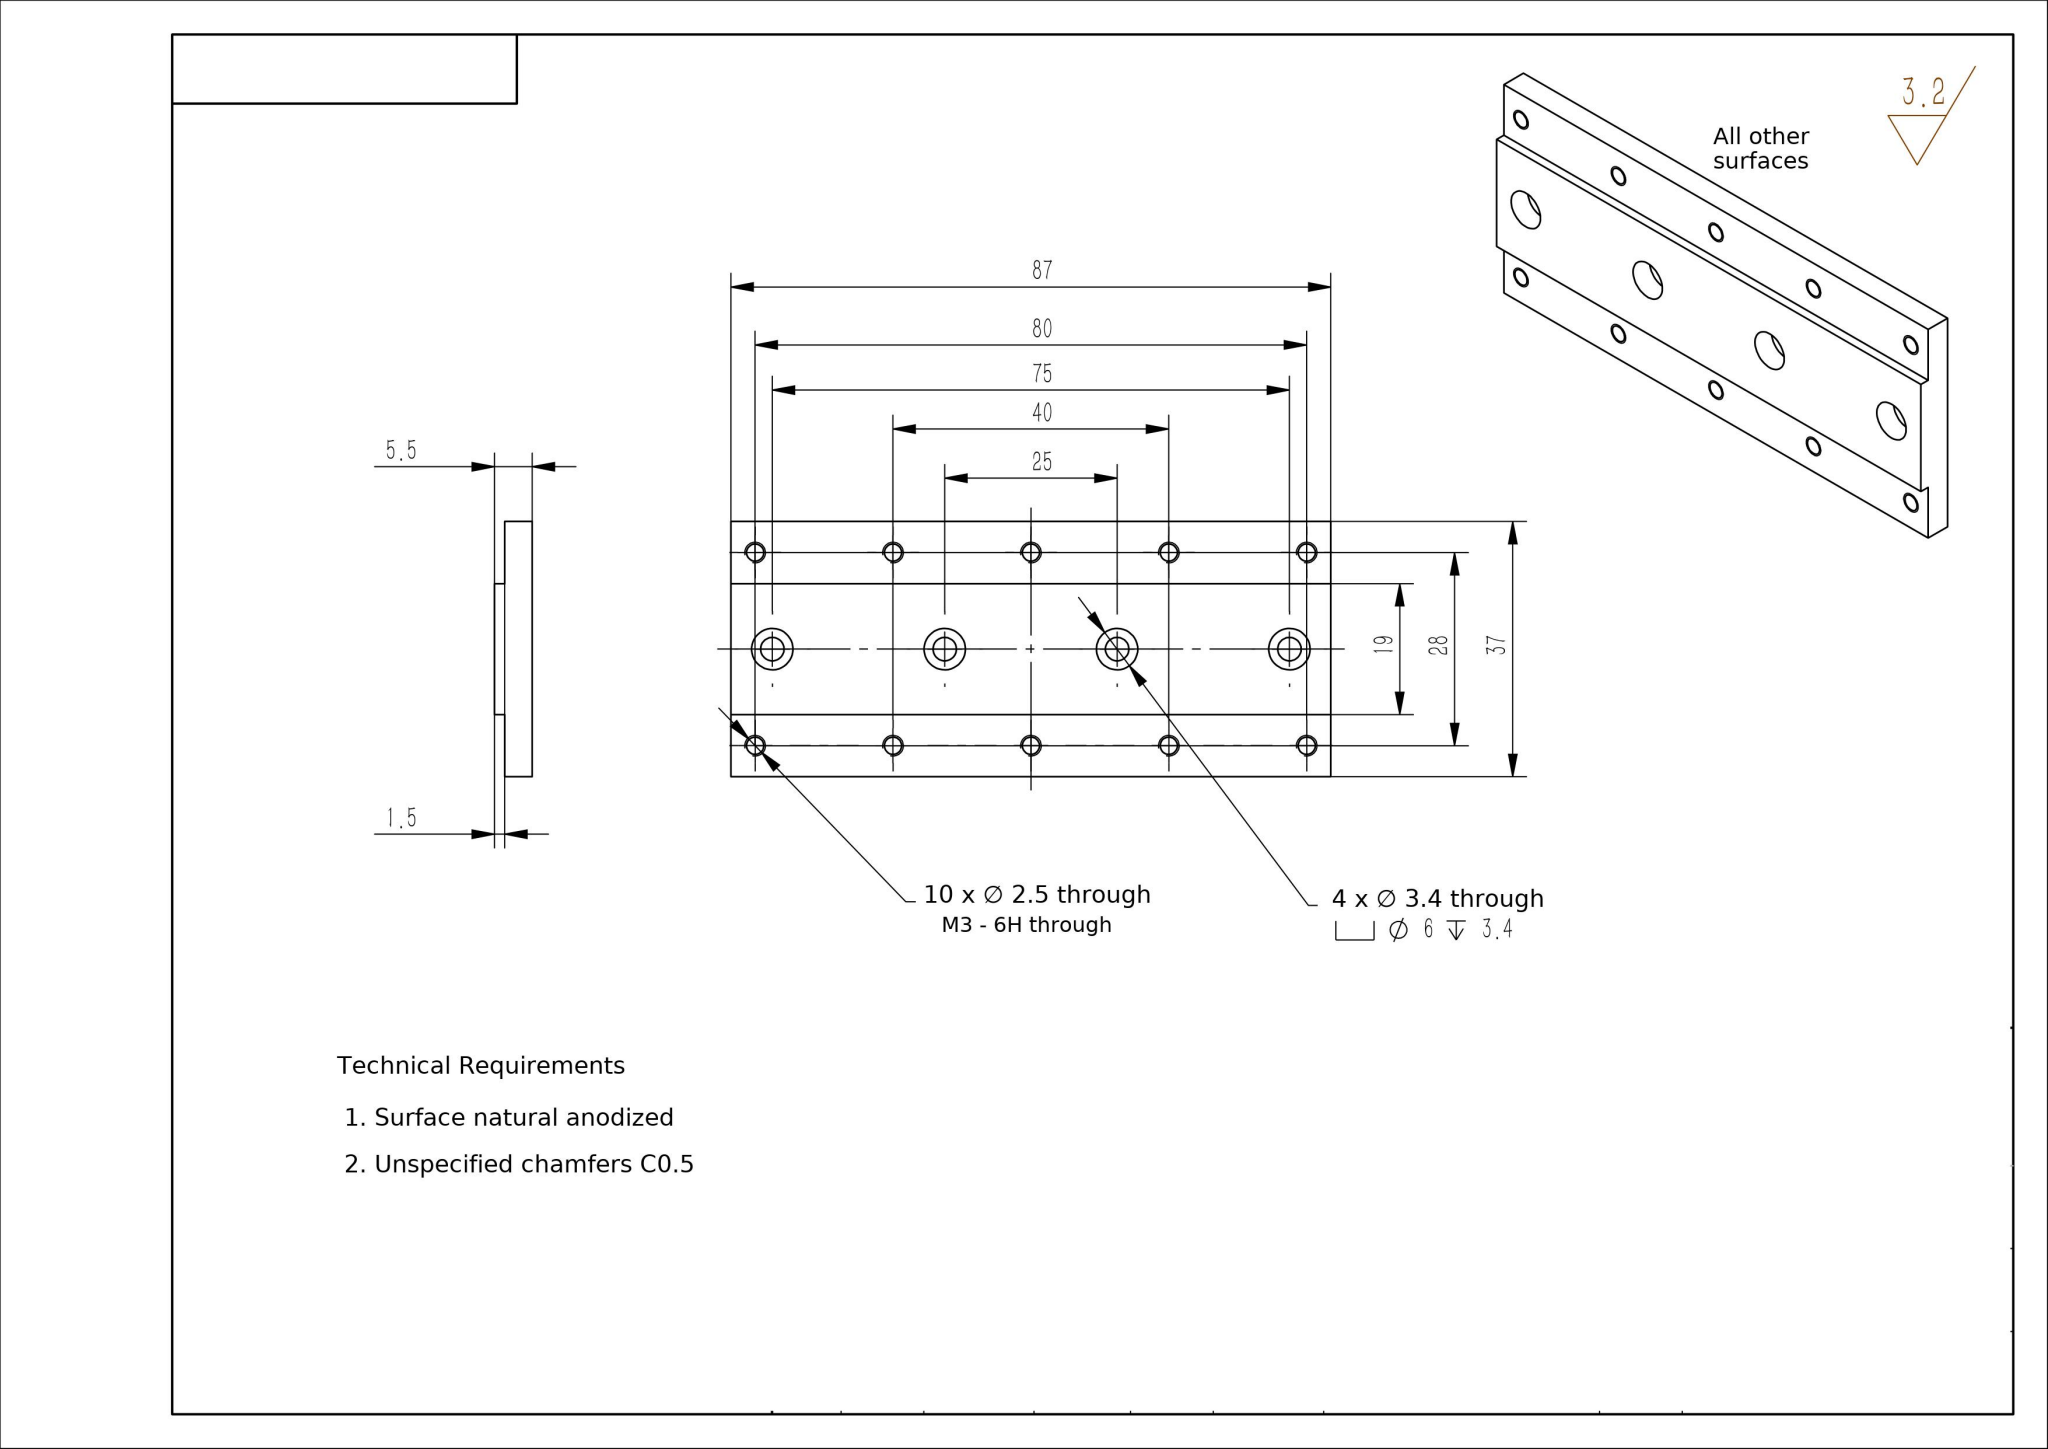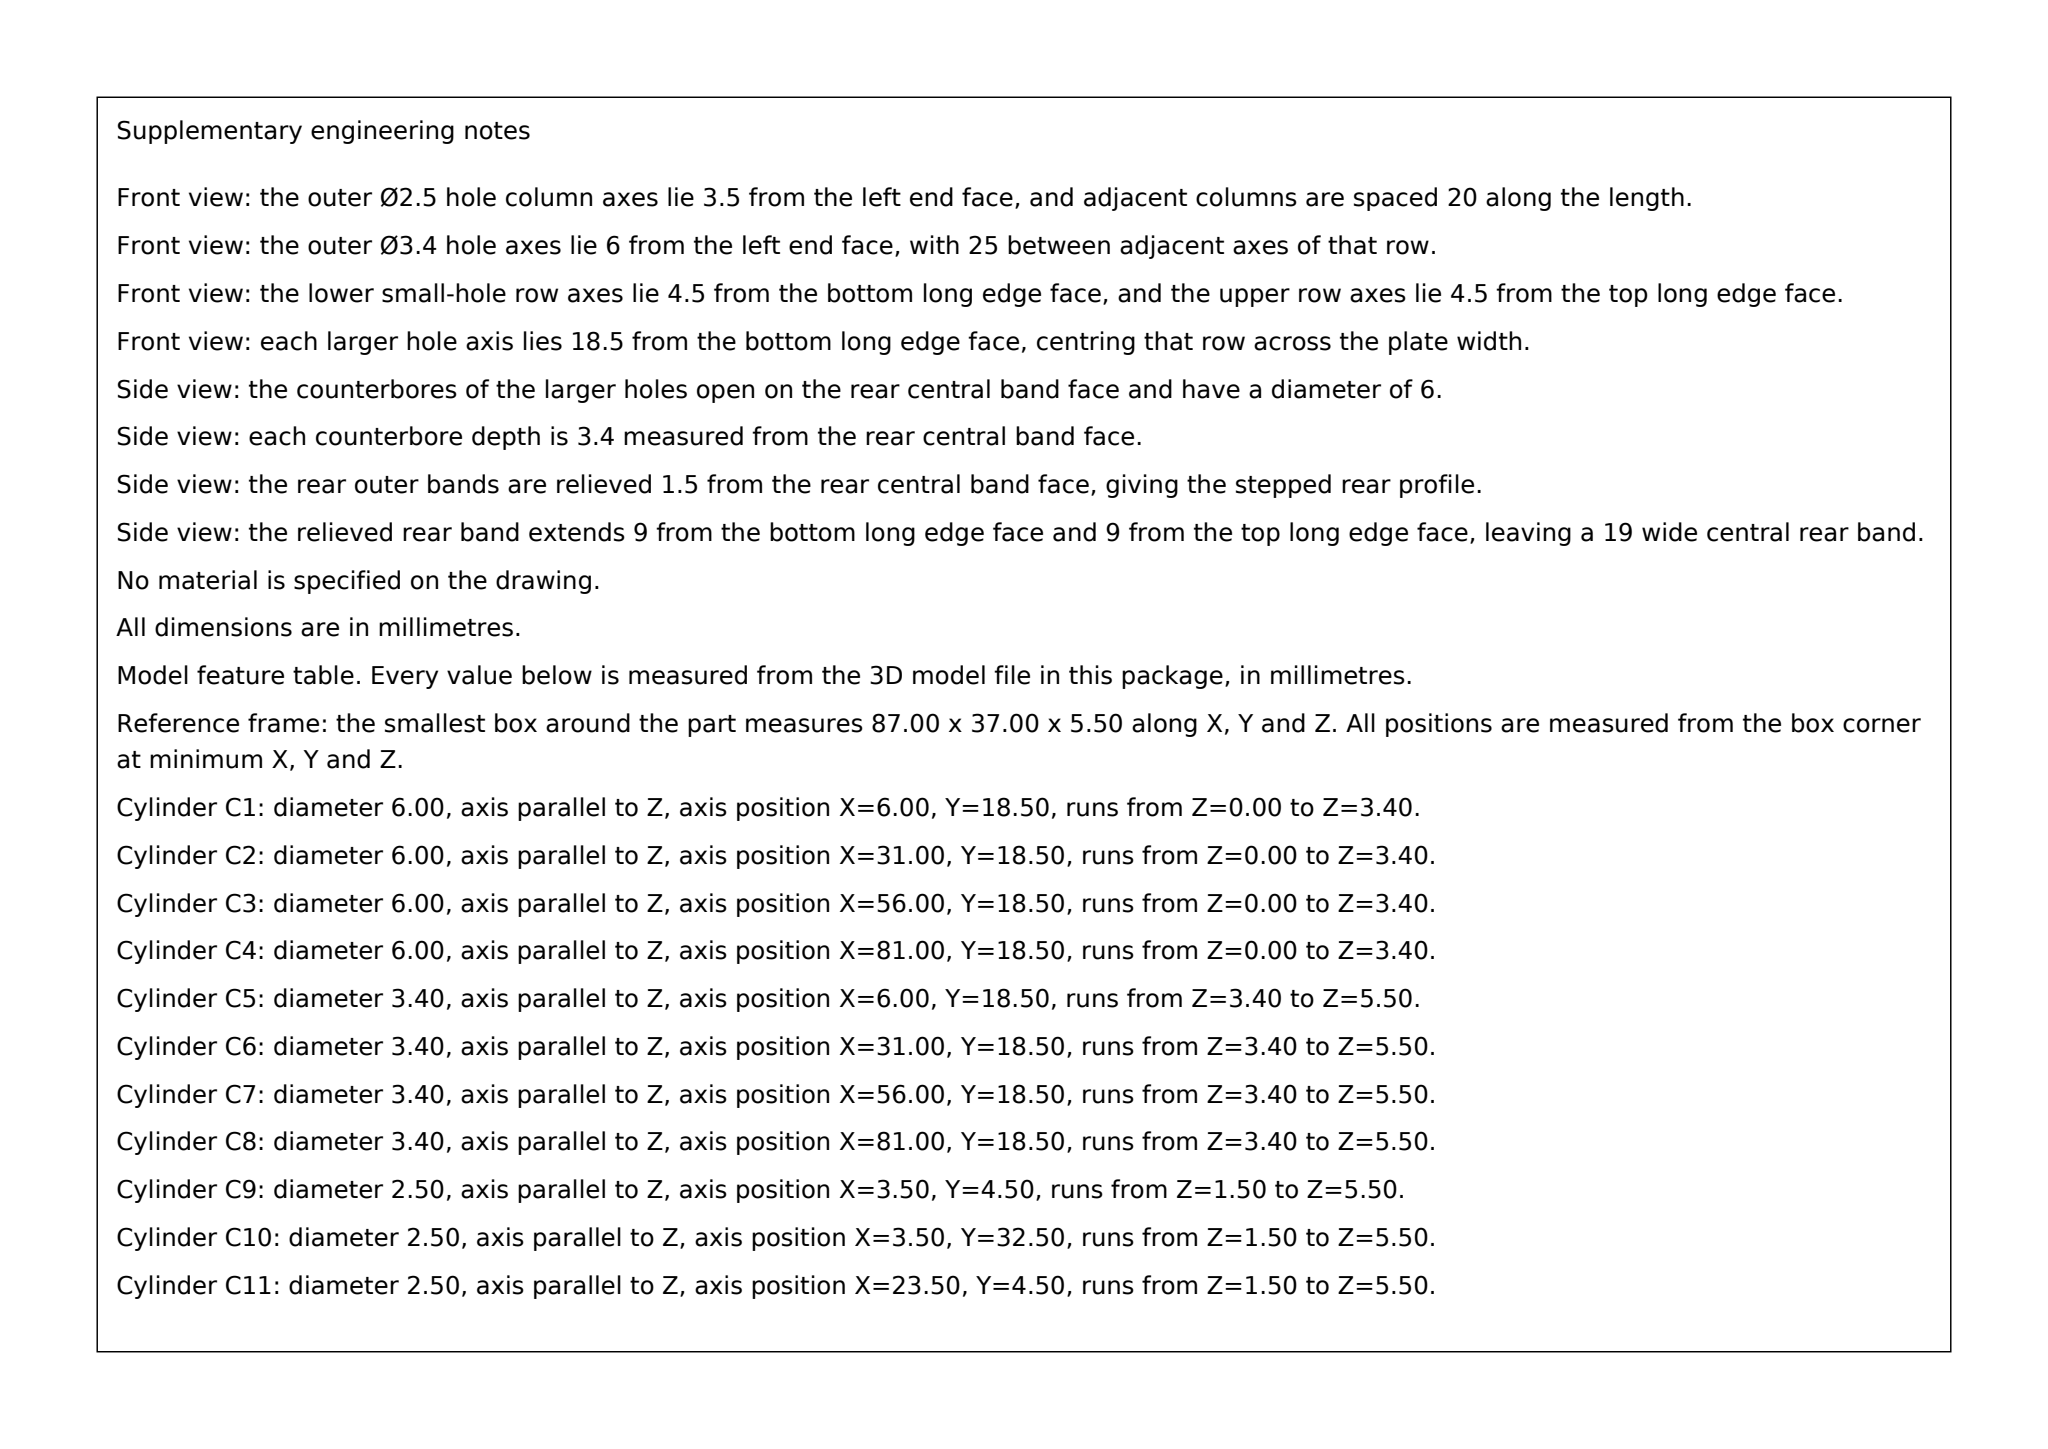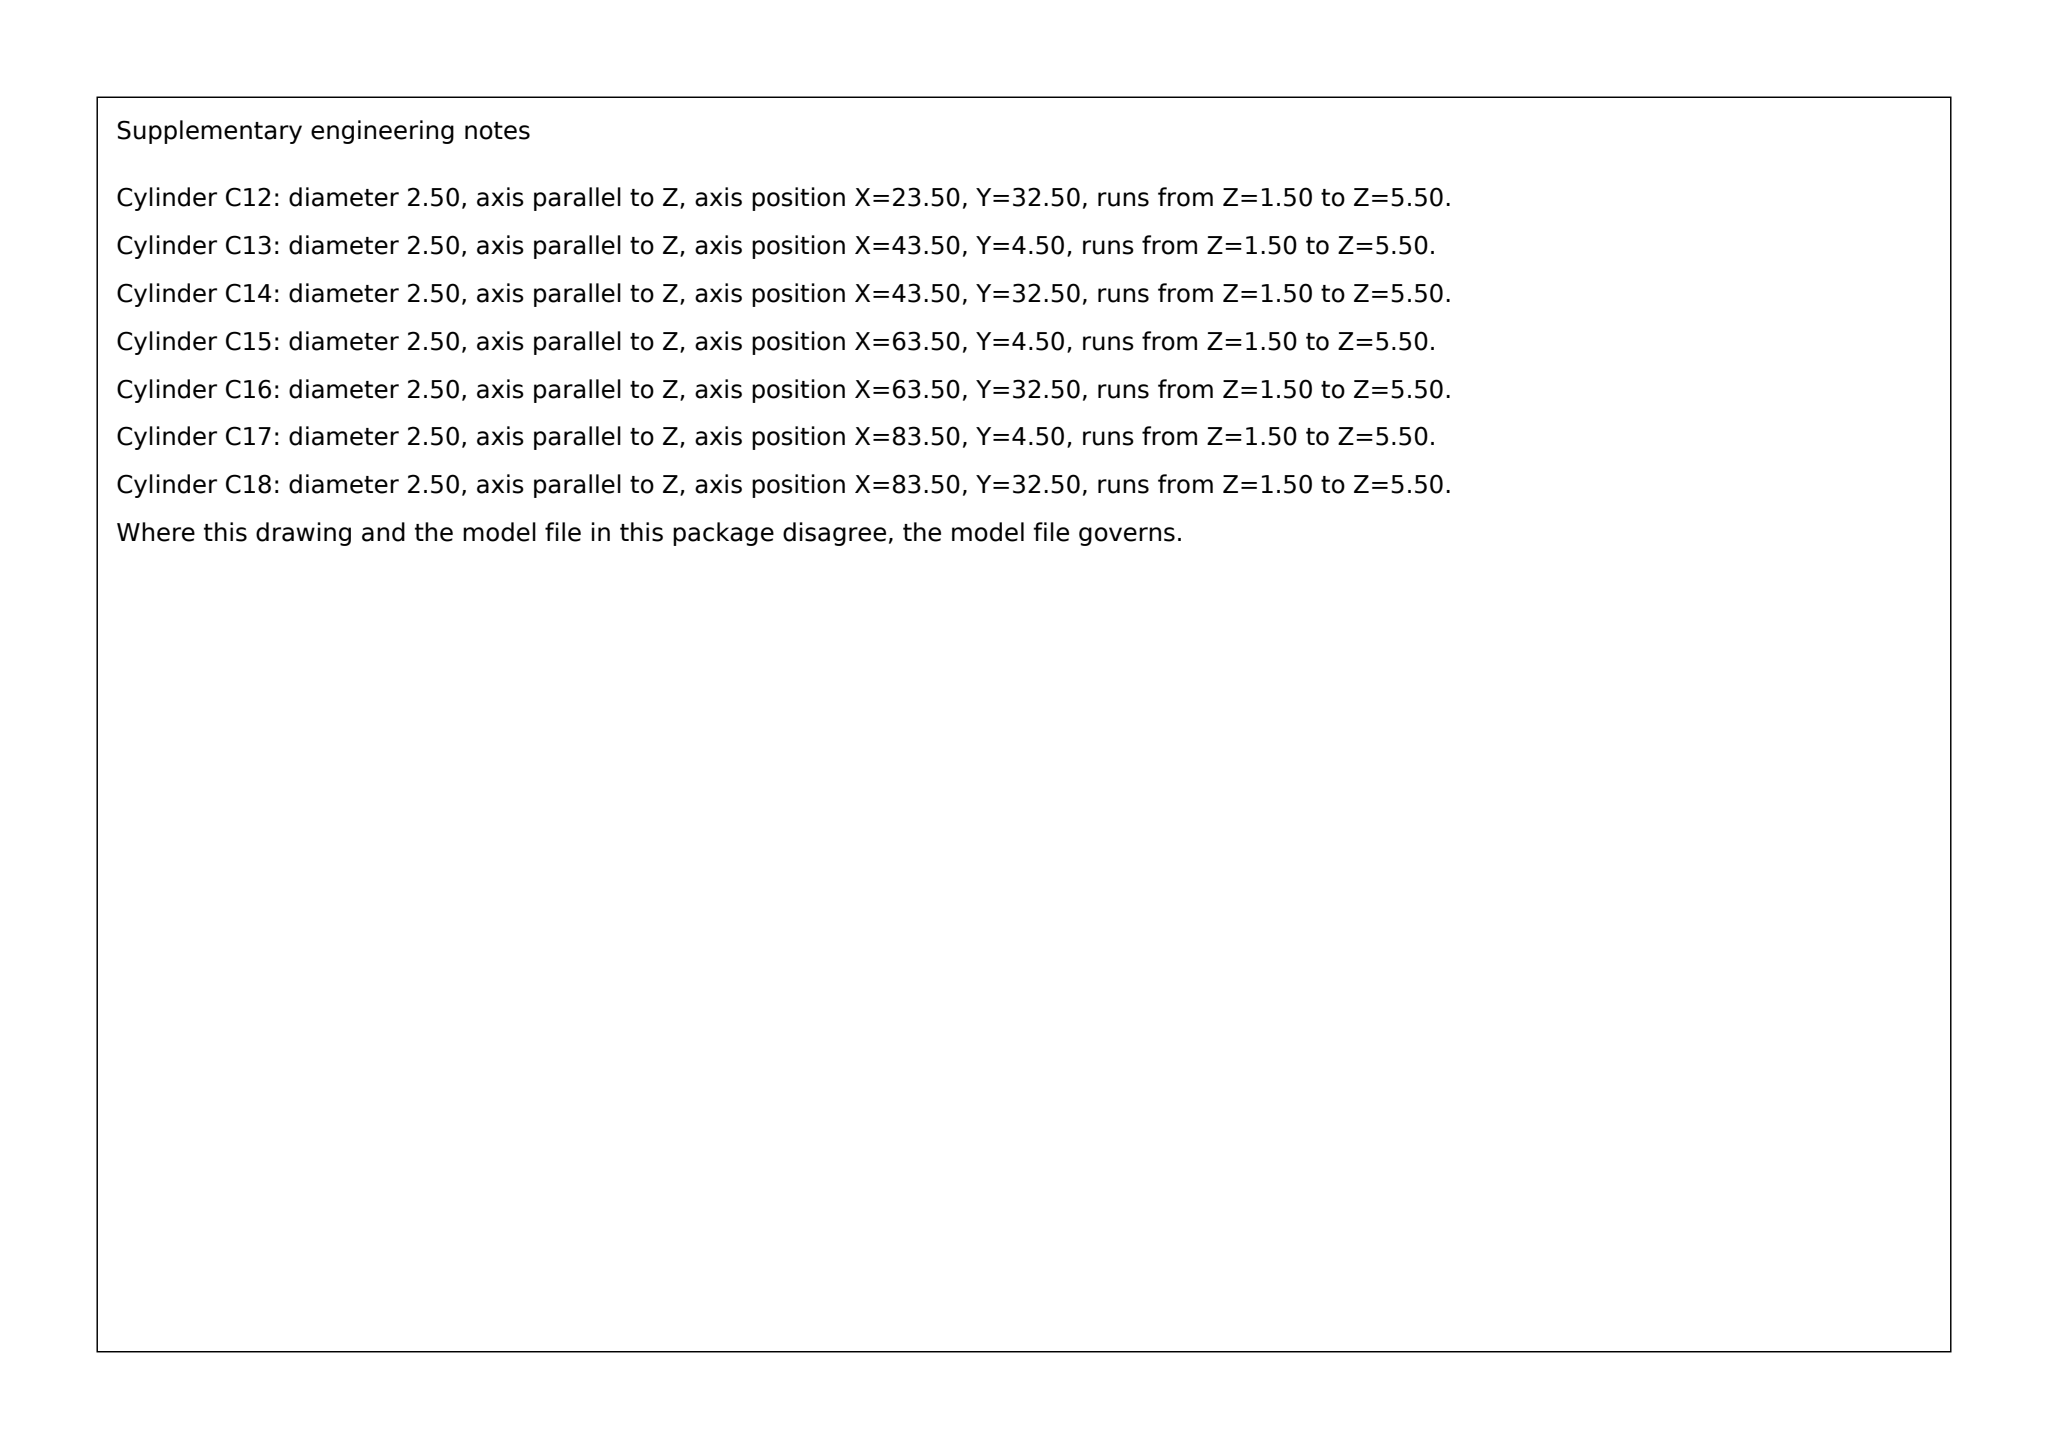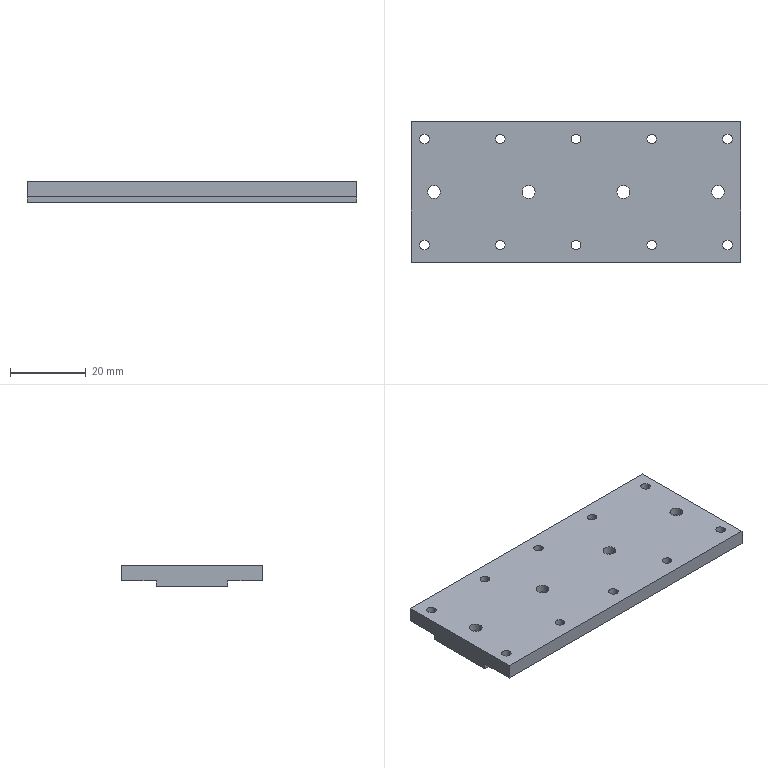Part | SolidWorks | mm | 1 solid | 50 faces | box 87 x 37 x 5.5 mm | volume 14698 mm3 | cylinder 36 | plane 14 | commonest cylinder face diameters 2.5 x20 6 x8 3.4 x8
Drawing notes:
CORNER M3 HOLES: 3.5 FROM END EDGE, 4.5 FROM LONG EDGES | from the solid: Ø2.5 thru holes at x=3.5 & 83.5 (bbox 87 long), y=4.5 & 32.5 (bbox 37 wide)
build123d program:
from build123d import *

# Parameters (mm, degrees)
SKETCH1_W                                         = 87
SKETCH1_H                                         = 5.5
BOSS_EXTRUDE1_DEPTH                               = 37
SKETCH3_W                                         = 87
SKETCH3_H                                         = 9
CUT_EXTRUDE2_DEPTH                                = 1.5
M3_TAPPED_HOLE2_D                                 = 2.5
LPATTERN1_COUNT                                   = 5
LPATTERN1_PITCH                                   = 20
MIRROR1_COPY_1_D                                  = 2.5
MIRROR1_COPY_2_D                                  = 2.5
MIRROR1_COPY_3_D                                  = 2.5
MIRROR1_COPY_4_D                                  = 2.5
HOLE_SIZE_ACCORDING_TO_HEXAGON_SOCKET_D           = 3.4
HOLE_SIZE_ACCORDING_TO_HEXAGON_SOCKET_CBORE_D     = 6
HOLE_SIZE_ACCORDING_TO_HEXAGON_SOCKET_CBORE_DEPTH = 3.4


with BuildPart() as part:
    # Sketch1 → Boss-Extrude1 (new body)
    with BuildSketch(Plane(origin=(0, 0, 0), x_dir=(1, 0, 0), z_dir=(0, 1, 0))):
        Rectangle(SKETCH1_W, SKETCH1_H)
    extrude(amount=BOSS_EXTRUDE1_DEPTH)

    # Sketch3 → Cut-Extrude2 (cut)
    with BuildSketch(Plane(origin=(0, 0, -2.75), x_dir=(-1, 0, 0), z_dir=(0, 0, -1))):
        with Locations((0, 4.5)):
            Rectangle(SKETCH3_W, SKETCH3_H)
        with Locations((0, 32.5)):
            Rectangle(SKETCH3_W, SKETCH3_H)
    extrude(amount=-CUT_EXTRUDE2_DEPTH, mode=Mode.SUBTRACT)

    # M3 Tapped Hole2 (through all)
    with Locations(Plane(origin=(0, 0, -1.25), x_dir=(-1, 0, 0), z_dir=(0, 0, -1))):
        with Locations((-40, 4.5)):
            m3_tapped_hole2 = Hole(M3_TAPPED_HOLE2_D / 2)

    # LPattern1: M3 Tapped Hole2 ×5
    with Locations(*[(-i * LPATTERN1_PITCH, 0, 0) for i in range(1, LPATTERN1_COUNT)]):
        add(m3_tapped_hole2, mode=Mode.SUBTRACT)

    # Mirror1: M3 Tapped Hole2 across plane
    add(m3_tapped_hole2.mirror(Plane(origin=(0, 18.5, 0), x_dir=(0, 0, 1), z_dir=(0, -1, 0))), mode=Mode.SUBTRACT)

    # Mirror1 copy 1 (through all)
    with Locations(Plane(origin=(-20, 37, -1.25), x_dir=(-1, 0, 0), z_dir=(0, 0, -1))):
        with Locations((-40, -4.5)):
            Hole(MIRROR1_COPY_1_D / 2)

    # Mirror1 copy 2 (through all)
    with Locations(Plane(origin=(-40, 37, -1.25), x_dir=(-1, 0, 0), z_dir=(0, 0, -1))):
        with Locations((-40, -4.5)):
            Hole(MIRROR1_COPY_2_D / 2)

    # Mirror1 copy 3 (through all)
    with Locations(Plane(origin=(-60, 37, -1.25), x_dir=(-1, 0, 0), z_dir=(0, 0, -1))):
        with Locations((-40, -4.5)):
            Hole(MIRROR1_COPY_3_D / 2)

    # Mirror1 copy 4 (through all)
    with Locations(Plane(origin=(-80, 37, -1.25), x_dir=(-1, 0, 0), z_dir=(0, 0, -1))):
        with Locations((-40, -4.5)):
            Hole(MIRROR1_COPY_4_D / 2)

    # Hole Size _ according to_ Hexagon Socket (through all)
    with Locations(Plane(origin=(0, 0, -2.75), x_dir=(-1, 0, 0), z_dir=(0, 0, -1))):
        with Locations((-37.5, 18.5), (-12.5, 18.5)):
            hole_size_according_to_hexagon_socket = CounterBoreHole(HOLE_SIZE_ACCORDING_TO_HEXAGON_SOCKET_D / 2, HOLE_SIZE_ACCORDING_TO_HEXAGON_SOCKET_CBORE_D / 2, HOLE_SIZE_ACCORDING_TO_HEXAGON_SOCKET_CBORE_DEPTH)

    # Mirror2: Hole Size _ according to_ Hexagon Socket across plane
    add(hole_size_according_to_hexagon_socket.mirror(Plane(origin=(0, 0, 0), x_dir=(0, 0, 1), z_dir=(1, 0, 0))), mode=Mode.SUBTRACT)


solid = part.part